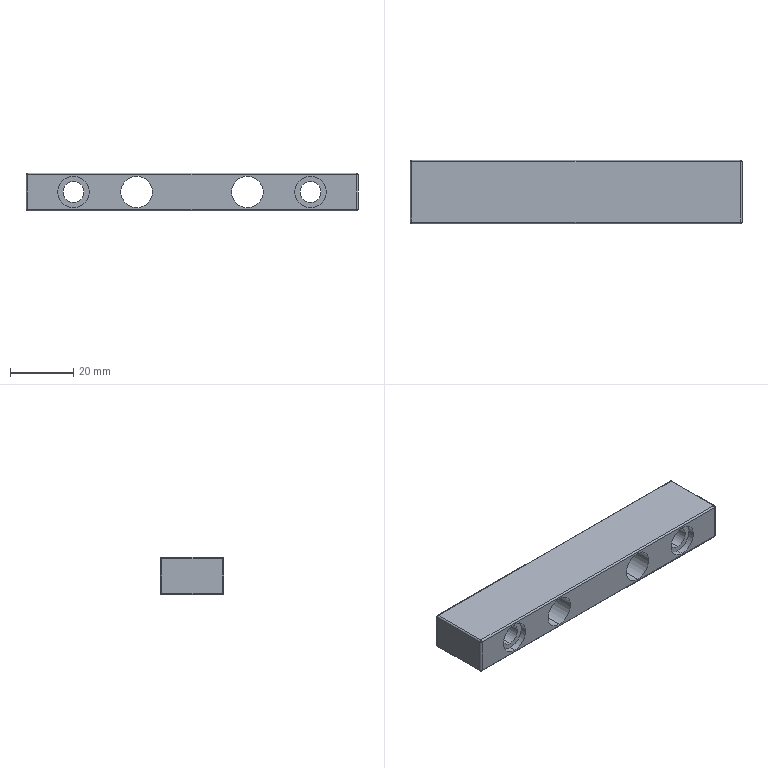Component | SolidWorks | F12529-M5104-1 | 1 solid | 48 faces | box 105 x 20 x 12 mm | volume 19267 mm3 | cylinder 28 | plane 12 | sphere 8 | commonest cylinder face diameters 1 x12 10 x8 11 x4 6.6 x4
build123d program:
from build123d import *

# Parameters (mm, degrees)
SKETCH1_W                                            = 105
SKETCH1_H                                            = 20
EXTRUDE1_DEPTH                                       = 6
FILLET1_R                                            = 0.5
SKETCH2_R                                            = 5
CUT_EXTRUDE1_DEPTH                                   = 2
M6_HEX_SOCKET_HEAD_CAP_SCREW_COUNTERBORE_D           = 6.6
M6_HEX_SOCKET_HEAD_CAP_SCREW_COUNTERBORE_CBORE_D     = 11
M6_HEX_SOCKET_HEAD_CAP_SCREW_COUNTERBORE_CBORE_DEPTH = 10
SKETCH5_R                                            = 5
CUT_EXTRUDE2_DEPTH                                   = 108.056


with BuildPart() as part:
    # Sketch1 → Extrude1 (new, symmetric)
    with BuildSketch(Plane.XY):
        with Locations((52.5, 10)):
            Rectangle(SKETCH1_W, SKETCH1_H)
    extrude(amount=EXTRUDE1_DEPTH, both=True)

    # Fillet1
    fillet1_edges = [part.edges().sort_by_distance(p)[0] for p in [
        (105, 10, 6),
        (52.5, 20, 6),
        (0, 10, 6),
        (52.5, 20, -6),
        (105, 10, -6),
        (52.5, 0, -6),
        (0, 10, -6),
        (52.5, 0, 6),
        (0, 20, 0),
        (105, 20, 0),
        (105, 0, 0),
        (0, 0, 0),
    ]]
    fillet(fillet1_edges, radius=FILLET1_R)

    # Sketch2 → Cut-Extrude1 (cut)
    with BuildSketch(Plane.XZ):
        with Locations(Location((15, 0, 0), (0, 0, 270))):
            Circle(SKETCH2_R)
        with Locations(Location((90, 0, 0), (0, 0, 270))):
            Circle(SKETCH2_R)
    extrude(amount=-CUT_EXTRUDE1_DEPTH, mode=Mode.SUBTRACT)

    # M6 Hex Socket Head Cap Screw Counterbore (through all)
    with Locations(Plane(origin=(0, 20, 0), x_dir=(-1, 0, 0), z_dir=(0, 1, 0))):
        with Locations((-90, 0), (-15, 0)):
            CounterBoreHole(M6_HEX_SOCKET_HEAD_CAP_SCREW_COUNTERBORE_D / 2, M6_HEX_SOCKET_HEAD_CAP_SCREW_COUNTERBORE_CBORE_D / 2, M6_HEX_SOCKET_HEAD_CAP_SCREW_COUNTERBORE_CBORE_DEPTH)

    # Sketch5 → Cut-Extrude2 (cut, through all)
    with BuildSketch(Plane(origin=(0, 20, 0), x_dir=(1, 0, 0), z_dir=(0, 1, 0))):
        with Locations(Location((35, 0, 0), (0, 0, 270))):
            Circle(SKETCH5_R)
        with Locations(Location((70, 0, 0), (0, 0, 270))):
            Circle(SKETCH5_R)
    extrude(amount=-CUT_EXTRUDE2_DEPTH, mode=Mode.SUBTRACT)


solid = part.part

# Placed as in the assembly
solid = solid.moved(Location((-52.5, 273, 10), (0, 0, 0)))